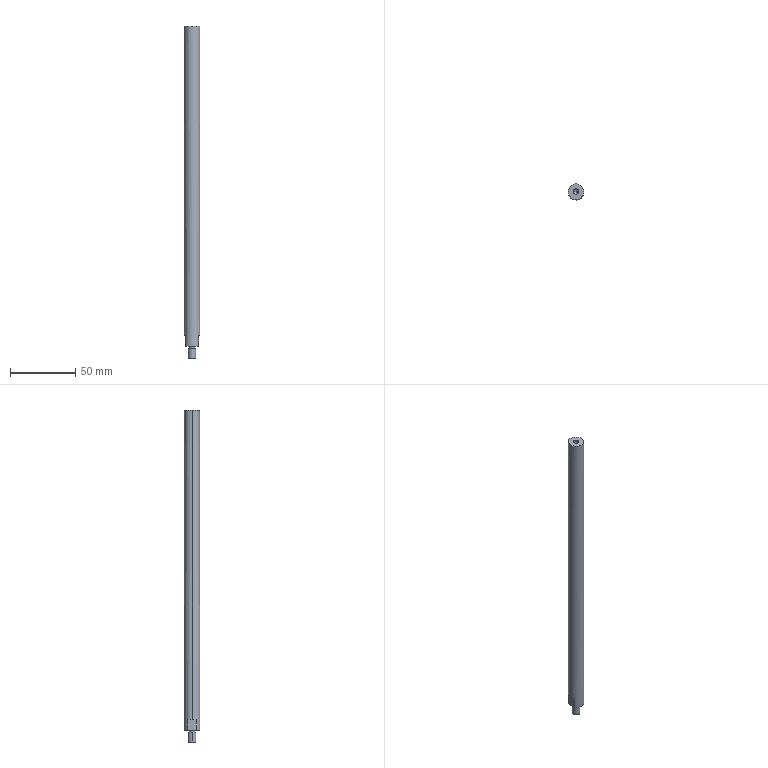CAM job | Mastercam | mm | 2 operations | part box 12 x 12 x 254
1. Contour (2D) | 14 - 12 平铣刀
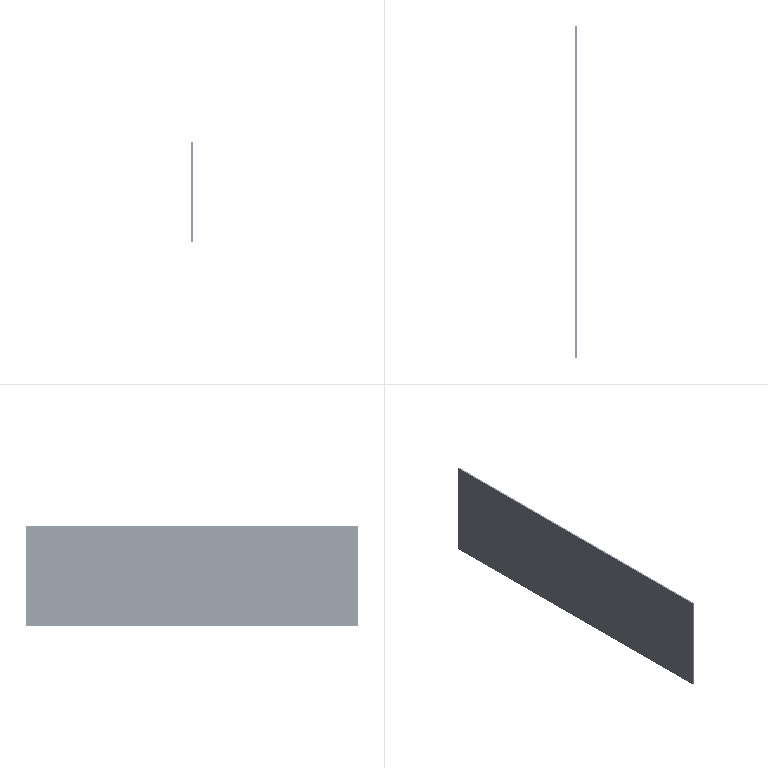2. Contour (2D) | 14 - 12 平铣刀